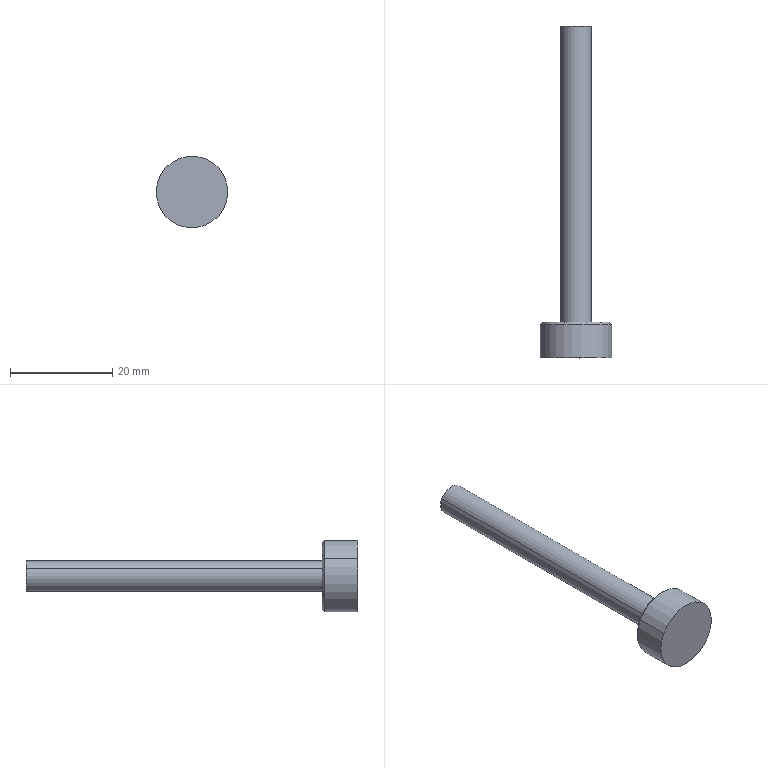Component | SolidWorks | GbgbMagnetPressingHead1F8-1 | 1 solid | 13 faces | box 14 x 65 x 14 mm | volume 2623 mm3 | cylinder 6 | cone 4 | plane 3 | commonest cylinder face diameters 14 x2 6 x2 3.3 x2
build123d program:
from build123d import *

# Parameters (mm, degrees)
SKETCH1_R             = 7
BOSS_EXTRUDE1_DEPTH   = 32.5
M4_TAPPED_HOLE1_D     = 3.3
M4_TAPPED_HOLE1_DEPTH = 10.1
M4_TAPPED_HOLE1_TIP   = 0.9914
SKETCH5_OUTSIDE_W     = 29.59
SKETCH5_OUTSIDE_H     = 29.59
SKETCH5_OUTSIDE_R     = 3
CUT_EXTRUDE2_DEPTH    = 58
CHAMFER2_SIZE         = 0.5


with BuildPart() as part:
    # Sketch1 → Boss-Extrude1 (new, symmetric)
    with BuildSketch(Plane(origin=(0, 0, 0), x_dir=(1, 0, 0), z_dir=(0, 1, 0))):
        with Locations(Location((0, 0, 0), (0, 0, 270))):
            Circle(SKETCH1_R)
    extrude(amount=BOSS_EXTRUDE1_DEPTH, both=True)

    # M4 Tapped Hole1
    with Locations(Plane(origin=(0, 32.5, 0), x_dir=(1, 0, 0), z_dir=(0, 1, 0))):
        with Locations((0, 0)):
            Hole(M4_TAPPED_HOLE1_D / 2, depth=M4_TAPPED_HOLE1_DEPTH)
            with Locations((0, 0, -(M4_TAPPED_HOLE1_DEPTH + M4_TAPPED_HOLE1_TIP / 2))):  # 118° drill point
                Cone(0, M4_TAPPED_HOLE1_D / 2, M4_TAPPED_HOLE1_TIP, mode=Mode.SUBTRACT)

    # Sketch5 outside → Cut-Extrude2 (cut)
    with BuildSketch(Plane(origin=(0, 32.5, 0), x_dir=(1, 0, 0), z_dir=(0, 1, 0))):
        Rectangle(SKETCH5_OUTSIDE_W, SKETCH5_OUTSIDE_H)
        with Locations(Location((0, 0, 0), (0, 0, 270))):
            Circle(SKETCH5_OUTSIDE_R, mode=Mode.SUBTRACT)
    extrude(amount=-CUT_EXTRUDE2_DEPTH, mode=Mode.SUBTRACT)

    # Chamfer2
    chamfer2_edges = [part.edges().sort_by_distance(p)[0] for p in [
        (0, -25.5, -7),
    ]]
    chamfer(chamfer2_edges, length=CHAMFER2_SIZE)


solid = part.part

# Placed as in the assembly
solid = solid.moved(Location((55.446, 389.592, 430.232), (0, 0, 0)))
STEP:
#1=COLOUR_RGB('',0.7922,0.8196,0.9333);
#2=FILL_AREA_STYLE_COLOUR('',#1);
#3=FILL_AREA_STYLE('',(#2));
#4=SURFACE_STYLE_FILL_AREA(#3);
#5=SURFACE_SIDE_STYLE('',(#4));
#6=SURFACE_STYLE_USAGE(.BOTH.,#5);
#7=PRESENTATION_STYLE_ASSIGNMENT((#6));
#8=CARTESIAN_POINT('',(2.408,14.334,16.816));
#9=VERTEX_POINT('',#8);
#10=CARTESIAN_POINT('',(1.958,14.334,17.061));
#11=VERTEX_POINT('',#10);
#12=CARTESIAN_POINT('',(2.183,14.334,16.938));
#13=DIRECTION('',(-0.,1.,0.));
#14=DIRECTION('',(0.8776,0.,-0.4794));
#15=AXIS2_PLACEMENT_3D('',#12,#13,#14);
#16=CIRCLE('',#15,0.2559);
#17=EDGE_CURVE('',#9,#11,#16,.T.);
#18=ORIENTED_EDGE('',*,*,#17,.F.);
#19=CARTESIAN_POINT('',(2.425,14.315,16.806));
#20=VERTEX_POINT('',#19);
#21=CARTESIAN_POINT('',(2.408,14.334,16.816));
#22=DIRECTION('',(0.6205,-0.7071,-0.339));
#23=VECTOR('',#22,39.37);
#24=LINE('',#21,#23);
#25=EDGE_CURVE('',#9,#20,#24,.T.);
#26=ORIENTED_EDGE('',*,*,#25,.T.);
#27=CARTESIAN_POINT('',(1.941,14.315,17.07));
#28=VERTEX_POINT('',#27);
#29=CARTESIAN_POINT('',(2.183,14.315,16.938));
#30=DIRECTION('',(0.,-1.,-0.));
#31=DIRECTION('',(0.8776,0.,-0.4794));
#32=AXIS2_PLACEMENT_3D('',#29,#30,#31);
#33=CIRCLE('',#32,0.2756);
#34=EDGE_CURVE('',#28,#20,#33,.T.);
#35=ORIENTED_EDGE('',*,*,#34,.F.);
#36=CARTESIAN_POINT('',(1.958,14.334,17.061));
#37=DIRECTION('',(-0.6205,-0.7071,0.339));
#38=VECTOR('',#37,39.37);
#39=LINE('',#36,#38);
#40=EDGE_CURVE('',#11,#28,#39,.T.);
#41=ORIENTED_EDGE('',*,*,#40,.F.);
#42=EDGE_LOOP('',(#18,#26,#35,#41));
#43=FACE_OUTER_BOUND('',#42,.T.);
#44=CARTESIAN_POINT('',(2.183,14.334,16.938));
#45=DIRECTION('',(0.,-1.,-0.));
#46=DIRECTION('',(-0.8776,0.,0.4794));
#47=AXIS2_PLACEMENT_3D('',#44,#45,#46);
#48=CONICAL_SURFACE('',#47,0.2559,0.7854);
#49=ADVANCED_FACE('',(#43),#48,.T.);
#50=ORIENTED_EDGE('',*,*,#34,.T.);
#51=CARTESIAN_POINT('',(2.425,14.059,16.806));
#52=VERTEX_POINT('',#51);
#53=CARTESIAN_POINT('',(2.425,16.618,16.806));
#54=DIRECTION('',(0.,-1.,-0.));
#55=VECTOR('',#54,39.37);
#56=LINE('',#53,#55);
#57=EDGE_CURVE('',#20,#52,#56,.T.);
#58=ORIENTED_EDGE('',*,*,#57,.T.);
#59=CARTESIAN_POINT('',(1.941,14.059,17.07));
#60=VERTEX_POINT('',#59);
#61=CARTESIAN_POINT('',(2.183,14.059,16.938));
#62=DIRECTION('',(-0.,1.,0.));
#63=DIRECTION('',(0.8776,0.,-0.4794));
#64=AXIS2_PLACEMENT_3D('',#61,#62,#63);
#65=CIRCLE('',#64,0.2756);
#66=EDGE_CURVE('',#52,#60,#65,.T.);
#67=ORIENTED_EDGE('',*,*,#66,.T.);
#68=CARTESIAN_POINT('',(1.941,16.618,17.07));
#69=DIRECTION('',(0.,-1.,-0.));
#70=VECTOR('',#69,39.37);
#71=LINE('',#68,#70);
#72=EDGE_CURVE('',#28,#60,#71,.T.);
#73=ORIENTED_EDGE('',*,*,#72,.F.);
#74=EDGE_LOOP('',(#50,#58,#67,#73));
#75=FACE_OUTER_BOUND('',#74,.T.);
#76=CARTESIAN_POINT('',(2.183,16.618,16.938));
#77=DIRECTION('',(0.,-1.,-0.));
#78=DIRECTION('',(-0.8776,0.,0.4794));
#79=AXIS2_PLACEMENT_3D('',#76,#77,#78);
#80=CYLINDRICAL_SURFACE('',#79,0.2756);
#81=ADVANCED_FACE('',(#75),#80,.T.);
#82=CARTESIAN_POINT('',(2.287,14.334,16.882));
#83=VERTEX_POINT('',#82);
#84=CARTESIAN_POINT('',(2.079,14.334,16.995));
#85=VERTEX_POINT('',#84);
#86=CARTESIAN_POINT('',(2.183,14.334,16.938));
#87=DIRECTION('',(-0.,1.,0.));
#88=DIRECTION('',(0.8776,0.,-0.4794));
#89=AXIS2_PLACEMENT_3D('',#86,#87,#88);
#90=CIRCLE('',#89,0.1181);
#91=EDGE_CURVE('',#83,#85,#90,.T.);
#92=ORIENTED_EDGE('',*,*,#91,.T.);
#93=CARTESIAN_POINT('',(2.079,16.618,16.995));
#94=VERTEX_POINT('',#93);
#95=CARTESIAN_POINT('',(2.079,14.334,16.995));
#96=DIRECTION('',(-0.,1.,0.));
#97=VECTOR('',#96,39.37);
#98=LINE('',#95,#97);
#99=EDGE_CURVE('',#85,#94,#98,.T.);
#100=ORIENTED_EDGE('',*,*,#99,.T.);
#101=CARTESIAN_POINT('',(2.287,16.618,16.882));
#102=VERTEX_POINT('',#101);
#103=CARTESIAN_POINT('',(2.183,16.618,16.938));
#104=DIRECTION('',(-0.,1.,0.));
#105=DIRECTION('',(0.8776,0.,-0.4794));
#106=AXIS2_PLACEMENT_3D('',#103,#104,#105);
#107=CIRCLE('',#106,0.1181);
#108=EDGE_CURVE('',#102,#94,#107,.T.);
#109=ORIENTED_EDGE('',*,*,#108,.F.);
#110=CARTESIAN_POINT('',(2.287,14.334,16.882));
#111=DIRECTION('',(-0.,1.,0.));
#112=VECTOR('',#111,39.37);
#113=LINE('',#110,#112);
#114=EDGE_CURVE('',#83,#102,#113,.T.);
#115=ORIENTED_EDGE('',*,*,#114,.F.);
#116=EDGE_LOOP('',(#92,#100,#109,#115));
#117=FACE_OUTER_BOUND('',#116,.T.);
#118=CARTESIAN_POINT('',(2.183,14.334,16.938));
#119=DIRECTION('',(-0.,1.,0.));
#120=DIRECTION('',(0.8776,0.,-0.4794));
#121=AXIS2_PLACEMENT_3D('',#118,#119,#120);
#122=CYLINDRICAL_SURFACE('',#121,0.1181);
#123=ADVANCED_FACE('',(#117),#122,.T.);
#124=CARTESIAN_POINT('',(2.126,16.22,16.969));
#125=VERTEX_POINT('',#124);
#126=CARTESIAN_POINT('',(2.24,16.22,16.907));
#127=VERTEX_POINT('',#126);
#128=CARTESIAN_POINT('',(2.183,16.22,16.938));
#129=DIRECTION('',(-0.,1.,0.));
#130=DIRECTION('',(0.8776,0.,-0.4794));
#131=AXIS2_PLACEMENT_3D('',#128,#129,#130);
#132=CIRCLE('',#131,0.06496);
#133=EDGE_CURVE('',#125,#127,#132,.T.);
#134=ORIENTED_EDGE('',*,*,#133,.F.);
#135=CARTESIAN_POINT('',(2.126,16.618,16.969));
#136=VERTEX_POINT('',#135);
#137=CARTESIAN_POINT('',(2.126,16.618,16.969));
#138=DIRECTION('',(-0.,1.,0.));
#139=VECTOR('',#138,39.37);
#140=LINE('',#137,#139);
#141=EDGE_CURVE('',#125,#136,#140,.T.);
#142=ORIENTED_EDGE('',*,*,#141,.T.);
#143=CARTESIAN_POINT('',(2.24,16.618,16.907));
#144=VERTEX_POINT('',#143);
#145=CARTESIAN_POINT('',(2.183,16.618,16.938));
#146=DIRECTION('',(-0.,1.,0.));
#147=DIRECTION('',(0.8776,0.,-0.4794));
#148=AXIS2_PLACEMENT_3D('',#145,#146,#147);
#149=CIRCLE('',#148,0.06496);
#150=EDGE_CURVE('',#136,#144,#149,.T.);
#151=ORIENTED_EDGE('',*,*,#150,.T.);
#152=CARTESIAN_POINT('',(2.24,16.618,16.907));
#153=DIRECTION('',(-0.,1.,0.));
#154=VECTOR('',#153,39.37);
#155=LINE('',#152,#154);
#156=EDGE_CURVE('',#127,#144,#155,.T.);
#157=ORIENTED_EDGE('',*,*,#156,.F.);
#158=EDGE_LOOP('',(#134,#142,#151,#157));
#159=FACE_OUTER_BOUND('',#158,.T.);
#160=CARTESIAN_POINT('',(2.183,16.618,16.938));
#161=DIRECTION('',(-0.,1.,0.));
#162=DIRECTION('',(0.8776,0.,-0.4794));
#163=AXIS2_PLACEMENT_3D('',#160,#161,#162);
#164=CYLINDRICAL_SURFACE('',#163,0.06496);
#165=ADVANCED_FACE('',(#159),#164,.F.);
#166=CARTESIAN_POINT('',(2.183,16.181,16.938));
#167=VERTEX_POINT('',#166);
#168=CARTESIAN_POINT('',(2.24,16.22,16.907));
#169=DIRECTION('',(0.7522,0.515,-0.411));
#170=VECTOR('',#169,39.37);
#171=LINE('',#168,#170);
#172=EDGE_CURVE('',#167,#127,#171,.T.);
#173=ORIENTED_EDGE('',*,*,#172,.F.);
#174=CARTESIAN_POINT('',(2.126,16.22,16.969));
#175=DIRECTION('',(-0.7522,0.515,0.411));
#176=VECTOR('',#175,39.37);
#177=LINE('',#174,#176);
#178=EDGE_CURVE('',#167,#125,#177,.T.);
#179=ORIENTED_EDGE('',*,*,#178,.T.);
#180=ORIENTED_EDGE('',*,*,#133,.T.);
#181=EDGE_LOOP('',(#173,#179,#180));
#182=FACE_OUTER_BOUND('',#181,.T.);
#183=CARTESIAN_POINT('',(2.183,16.22,16.938));
#184=DIRECTION('',(-0.,1.,0.));
#185=DIRECTION('',(0.8776,0.,-0.4794));
#186=AXIS2_PLACEMENT_3D('',#183,#184,#185);
#187=CONICAL_SURFACE('',#186,0.06496,1.03);
#188=ADVANCED_FACE('',(#182),#187,.F.);
#189=CARTESIAN_POINT('',(2.183,16.618,16.938));
#190=DIRECTION('',(-0.,1.,0.));
#191=DIRECTION('',(0.8776,0.,-0.4794));
#192=AXIS2_PLACEMENT_3D('',#189,#190,#191);
#193=CIRCLE('',#192,0.06496);
#194=EDGE_CURVE('',#144,#136,#193,.T.);
#195=ORIENTED_EDGE('',*,*,#194,.F.);
#196=ORIENTED_EDGE('',*,*,#150,.F.);
#197=EDGE_LOOP('',(#195,#196));
#198=FACE_BOUND('',#197,.T.);
#199=ORIENTED_EDGE('',*,*,#108,.T.);
#200=CARTESIAN_POINT('',(2.183,16.618,16.938));
#201=DIRECTION('',(-0.,1.,0.));
#202=DIRECTION('',(0.8776,0.,-0.4794));
#203=AXIS2_PLACEMENT_3D('',#200,#201,#202);
#204=CIRCLE('',#203,0.1181);
#205=EDGE_CURVE('',#94,#102,#204,.T.);
#206=ORIENTED_EDGE('',*,*,#205,.T.);
#207=EDGE_LOOP('',(#199,#206));
#208=FACE_OUTER_BOUND('',#207,.T.);
#209=CARTESIAN_POINT('',(2.183,16.618,16.938));
#210=DIRECTION('',(-0.,1.,0.));
#211=DIRECTION('',(0.8776,0.,-0.4794));
#212=AXIS2_PLACEMENT_3D('',#209,#210,#211);
#213=PLANE('',#212);
#214=ADVANCED_FACE('',(#198,#208),#213,.T.);
#215=ORIENTED_EDGE('',*,*,#178,.F.);
#216=ORIENTED_EDGE('',*,*,#172,.T.);
#217=CARTESIAN_POINT('',(2.183,16.22,16.938));
#218=DIRECTION('',(-0.,1.,0.));
#219=DIRECTION('',(0.8776,0.,-0.4794));
#220=AXIS2_PLACEMENT_3D('',#217,#218,#219);
#221=CIRCLE('',#220,0.06496);
#222=EDGE_CURVE('',#127,#125,#221,.T.);
#223=ORIENTED_EDGE('',*,*,#222,.T.);
#224=EDGE_LOOP('',(#215,#216,#223));
#225=FACE_OUTER_BOUND('',#224,.T.);
#226=CARTESIAN_POINT('',(2.183,16.22,16.938));
#227=DIRECTION('',(-0.,1.,0.));
#228=DIRECTION('',(0.8776,0.,-0.4794));
#229=AXIS2_PLACEMENT_3D('',#226,#227,#228);
#230=CONICAL_SURFACE('',#229,0.06496,1.03);
#231=ADVANCED_FACE('',(#225),#230,.F.);
#232=ORIENTED_EDGE('',*,*,#141,.F.);
#233=ORIENTED_EDGE('',*,*,#222,.F.);
#234=ORIENTED_EDGE('',*,*,#156,.T.);
#235=ORIENTED_EDGE('',*,*,#194,.T.);
#236=EDGE_LOOP('',(#232,#233,#234,#235));
#237=FACE_OUTER_BOUND('',#236,.T.);
#238=CARTESIAN_POINT('',(2.183,16.618,16.938));
#239=DIRECTION('',(-0.,1.,0.));
#240=DIRECTION('',(0.8776,0.,-0.4794));
#241=AXIS2_PLACEMENT_3D('',#238,#239,#240);
#242=CYLINDRICAL_SURFACE('',#241,0.06496);
#243=ADVANCED_FACE('',(#237),#242,.F.);
#244=CARTESIAN_POINT('',(2.183,14.334,16.938));
#245=DIRECTION('',(-0.,1.,0.));
#246=DIRECTION('',(0.8776,0.,-0.4794));
#247=AXIS2_PLACEMENT_3D('',#244,#245,#246);
#248=CIRCLE('',#247,0.2559);
#249=EDGE_CURVE('',#11,#9,#248,.T.);
#250=ORIENTED_EDGE('',*,*,#249,.T.);
#251=ORIENTED_EDGE('',*,*,#17,.T.);
#252=EDGE_LOOP('',(#250,#251));
#253=FACE_OUTER_BOUND('',#252,.T.);
#254=ORIENTED_EDGE('',*,*,#91,.F.);
#255=CARTESIAN_POINT('',(2.183,14.334,16.938));
#256=DIRECTION('',(-0.,1.,0.));
#257=DIRECTION('',(0.8776,0.,-0.4794));
#258=AXIS2_PLACEMENT_3D('',#255,#256,#257);
#259=CIRCLE('',#258,0.1181);
#260=EDGE_CURVE('',#85,#83,#259,.T.);
#261=ORIENTED_EDGE('',*,*,#260,.F.);
#262=EDGE_LOOP('',(#254,#261));
#263=FACE_BOUND('',#262,.T.);
#264=CARTESIAN_POINT('',(2.183,14.334,16.938));
#265=DIRECTION('',(-0.,1.,0.));
#266=DIRECTION('',(0.8776,0.,-0.4794));
#267=AXIS2_PLACEMENT_3D('',#264,#265,#266);
#268=PLANE('',#267);
#269=ADVANCED_FACE('',(#253,#263),#268,.T.);
#270=ORIENTED_EDGE('',*,*,#99,.F.);
#271=ORIENTED_EDGE('',*,*,#260,.T.);
#272=ORIENTED_EDGE('',*,*,#114,.T.);
#273=ORIENTED_EDGE('',*,*,#205,.F.);
#274=EDGE_LOOP('',(#270,#271,#272,#273));
#275=FACE_OUTER_BOUND('',#274,.T.);
#276=CARTESIAN_POINT('',(2.183,14.334,16.938));
#277=DIRECTION('',(-0.,1.,0.));
#278=DIRECTION('',(0.8776,0.,-0.4794));
#279=AXIS2_PLACEMENT_3D('',#276,#277,#278);
#280=CYLINDRICAL_SURFACE('',#279,0.1181);
#281=ADVANCED_FACE('',(#275),#280,.T.);
#282=CARTESIAN_POINT('',(2.183,14.059,16.938));
#283=DIRECTION('',(-0.,1.,0.));
#284=DIRECTION('',(0.8776,0.,-0.4794));
#285=AXIS2_PLACEMENT_3D('',#282,#283,#284);
#286=CIRCLE('',#285,0.2756);
#287=EDGE_CURVE('',#60,#52,#286,.T.);
#288=ORIENTED_EDGE('',*,*,#287,.F.);
#289=ORIENTED_EDGE('',*,*,#66,.F.);
#290=EDGE_LOOP('',(#288,#289));
#291=FACE_OUTER_BOUND('',#290,.T.);
#292=CARTESIAN_POINT('',(2.183,14.059,16.938));
#293=DIRECTION('',(-0.,1.,0.));
#294=DIRECTION('',(0.8776,0.,-0.4794));
#295=AXIS2_PLACEMENT_3D('',#292,#293,#294);
#296=PLANE('',#295);
#297=ADVANCED_FACE('',(#291),#296,.F.);
#298=ORIENTED_EDGE('',*,*,#57,.F.);
#299=CARTESIAN_POINT('',(2.183,14.315,16.938));
#300=DIRECTION('',(0.,-1.,-0.));
#301=DIRECTION('',(0.8776,0.,-0.4794));
#302=AXIS2_PLACEMENT_3D('',#299,#300,#301);
#303=CIRCLE('',#302,0.2756);
#304=EDGE_CURVE('',#20,#28,#303,.T.);
#305=ORIENTED_EDGE('',*,*,#304,.T.);
#306=ORIENTED_EDGE('',*,*,#72,.T.);
#307=ORIENTED_EDGE('',*,*,#287,.T.);
#308=EDGE_LOOP('',(#298,#305,#306,#307));
#309=FACE_OUTER_BOUND('',#308,.T.);
#310=CARTESIAN_POINT('',(2.183,16.618,16.938));
#311=DIRECTION('',(0.,-1.,-0.));
#312=DIRECTION('',(-0.8776,0.,0.4794));
#313=AXIS2_PLACEMENT_3D('',#310,#311,#312);
#314=CYLINDRICAL_SURFACE('',#313,0.2756);
#315=ADVANCED_FACE('',(#309),#314,.T.);
#316=ORIENTED_EDGE('',*,*,#25,.F.);
#317=ORIENTED_EDGE('',*,*,#249,.F.);
#318=ORIENTED_EDGE('',*,*,#40,.T.);
#319=ORIENTED_EDGE('',*,*,#304,.F.);
#320=EDGE_LOOP('',(#316,#317,#318,#319));
#321=FACE_OUTER_BOUND('',#320,.T.);
#322=CARTESIAN_POINT('',(2.183,14.334,16.938));
#323=DIRECTION('',(0.,-1.,-0.));
#324=DIRECTION('',(-0.8776,0.,0.4794));
#325=AXIS2_PLACEMENT_3D('',#322,#323,#324);
#326=CONICAL_SURFACE('',#325,0.2559,0.7854);
#327=ADVANCED_FACE('',(#321),#326,.T.);
#328=CLOSED_SHELL('',(#49,#81,#123,#165,#188,#214,#231,#243,#269,#281,#297,#315,#327));
#329=MANIFOLD_SOLID_BREP('',#328);
#330=STYLED_ITEM('',(#7),#329);
#331=(LENGTH_UNIT()NAMED_UNIT(*)SI_UNIT($,.METRE.));
#332=LENGTH_MEASURE_WITH_UNIT(LENGTH_MEASURE(0.0254),#331);
#333=DIMENSIONAL_EXPONENTS(1.,0.,0.,0.,0.,0.,0.);
#334=(CONVERSION_BASED_UNIT('',#332)LENGTH_UNIT()NAMED_UNIT(#333));
#335=UNCERTAINTY_MEASURE_WITH_UNIT(LENGTH_MEASURE(0.00001),#334,'','');
#336=(NAMED_UNIT(*)PLANE_ANGLE_UNIT()SI_UNIT($,.RADIAN.));
#337=(NAMED_UNIT(*)SI_UNIT($,.STERADIAN.)SOLID_ANGLE_UNIT());
#338=(GEOMETRIC_REPRESENTATION_CONTEXT(3)GLOBAL_UNCERTAINTY_ASSIGNED_CONTEXT((#335))GLOBAL_UNIT_ASSIGNED_CONTEXT((#334,#336,#337))REPRESENTATION_CONTEXT('',''));
#339=MECHANICAL_DESIGN_GEOMETRIC_PRESENTATION_REPRESENTATION('',(#330),#338);
#340=CARTESIAN_POINT('',(0.,0.,0.));
#341=DIRECTION('',(0.,0.,1.));
#342=DIRECTION('',(1.,0.,0.));
#343=AXIS2_PLACEMENT_3D('',#340,#341,#342);
#344=(LENGTH_UNIT()NAMED_UNIT(*)SI_UNIT($,.METRE.));
#345=LENGTH_MEASURE_WITH_UNIT(LENGTH_MEASURE(0.0254),#344);
#346=DIMENSIONAL_EXPONENTS(1.,0.,0.,0.,0.,0.,0.);
#347=(CONVERSION_BASED_UNIT('',#345)LENGTH_UNIT()NAMED_UNIT(#346));
#348=UNCERTAINTY_MEASURE_WITH_UNIT(LENGTH_MEASURE(0.00001),#347,'','');
#349=(NAMED_UNIT(*)PLANE_ANGLE_UNIT()SI_UNIT($,.RADIAN.));
#350=(NAMED_UNIT(*)SI_UNIT($,.STERADIAN.)SOLID_ANGLE_UNIT());
#351=(GEOMETRIC_REPRESENTATION_CONTEXT(3)GLOBAL_UNCERTAINTY_ASSIGNED_CONTEXT((#348))GLOBAL_UNIT_ASSIGNED_CONTEXT((#347,#349,#350))REPRESENTATION_CONTEXT('',''));
#352=ADVANCED_BREP_SHAPE_REPRESENTATION('',(#329,#343),#351);
#353=PRESENTATION_LAYER_ASSIGNMENT('','',(#330));